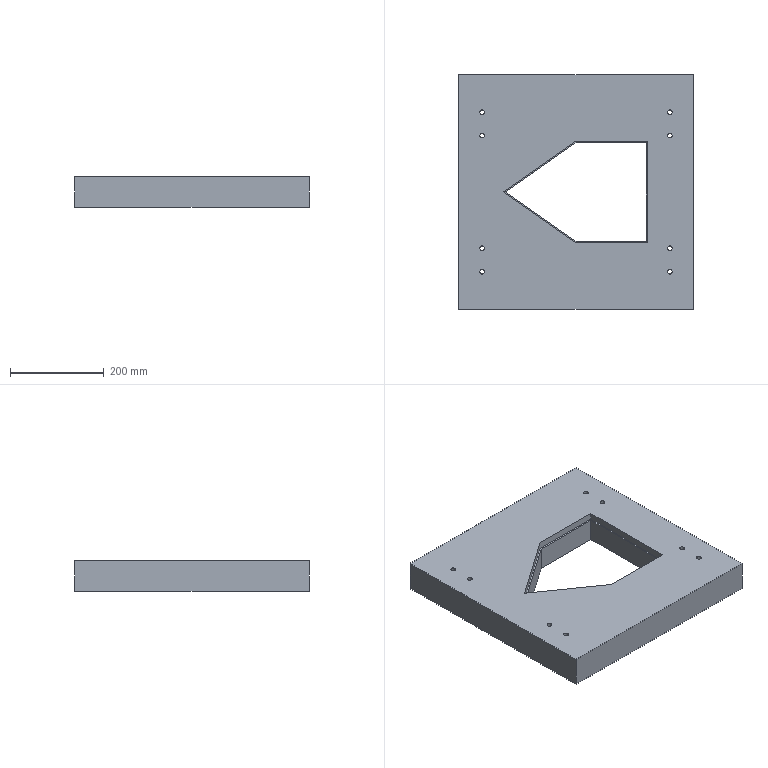Component | NX | DIE | 1 solid | 33 faces | volume 13099010 mm3 | plane 17 | cylinder 8 | cone 8 | commonest cylinder face diameters 9.732 x4 10 x4